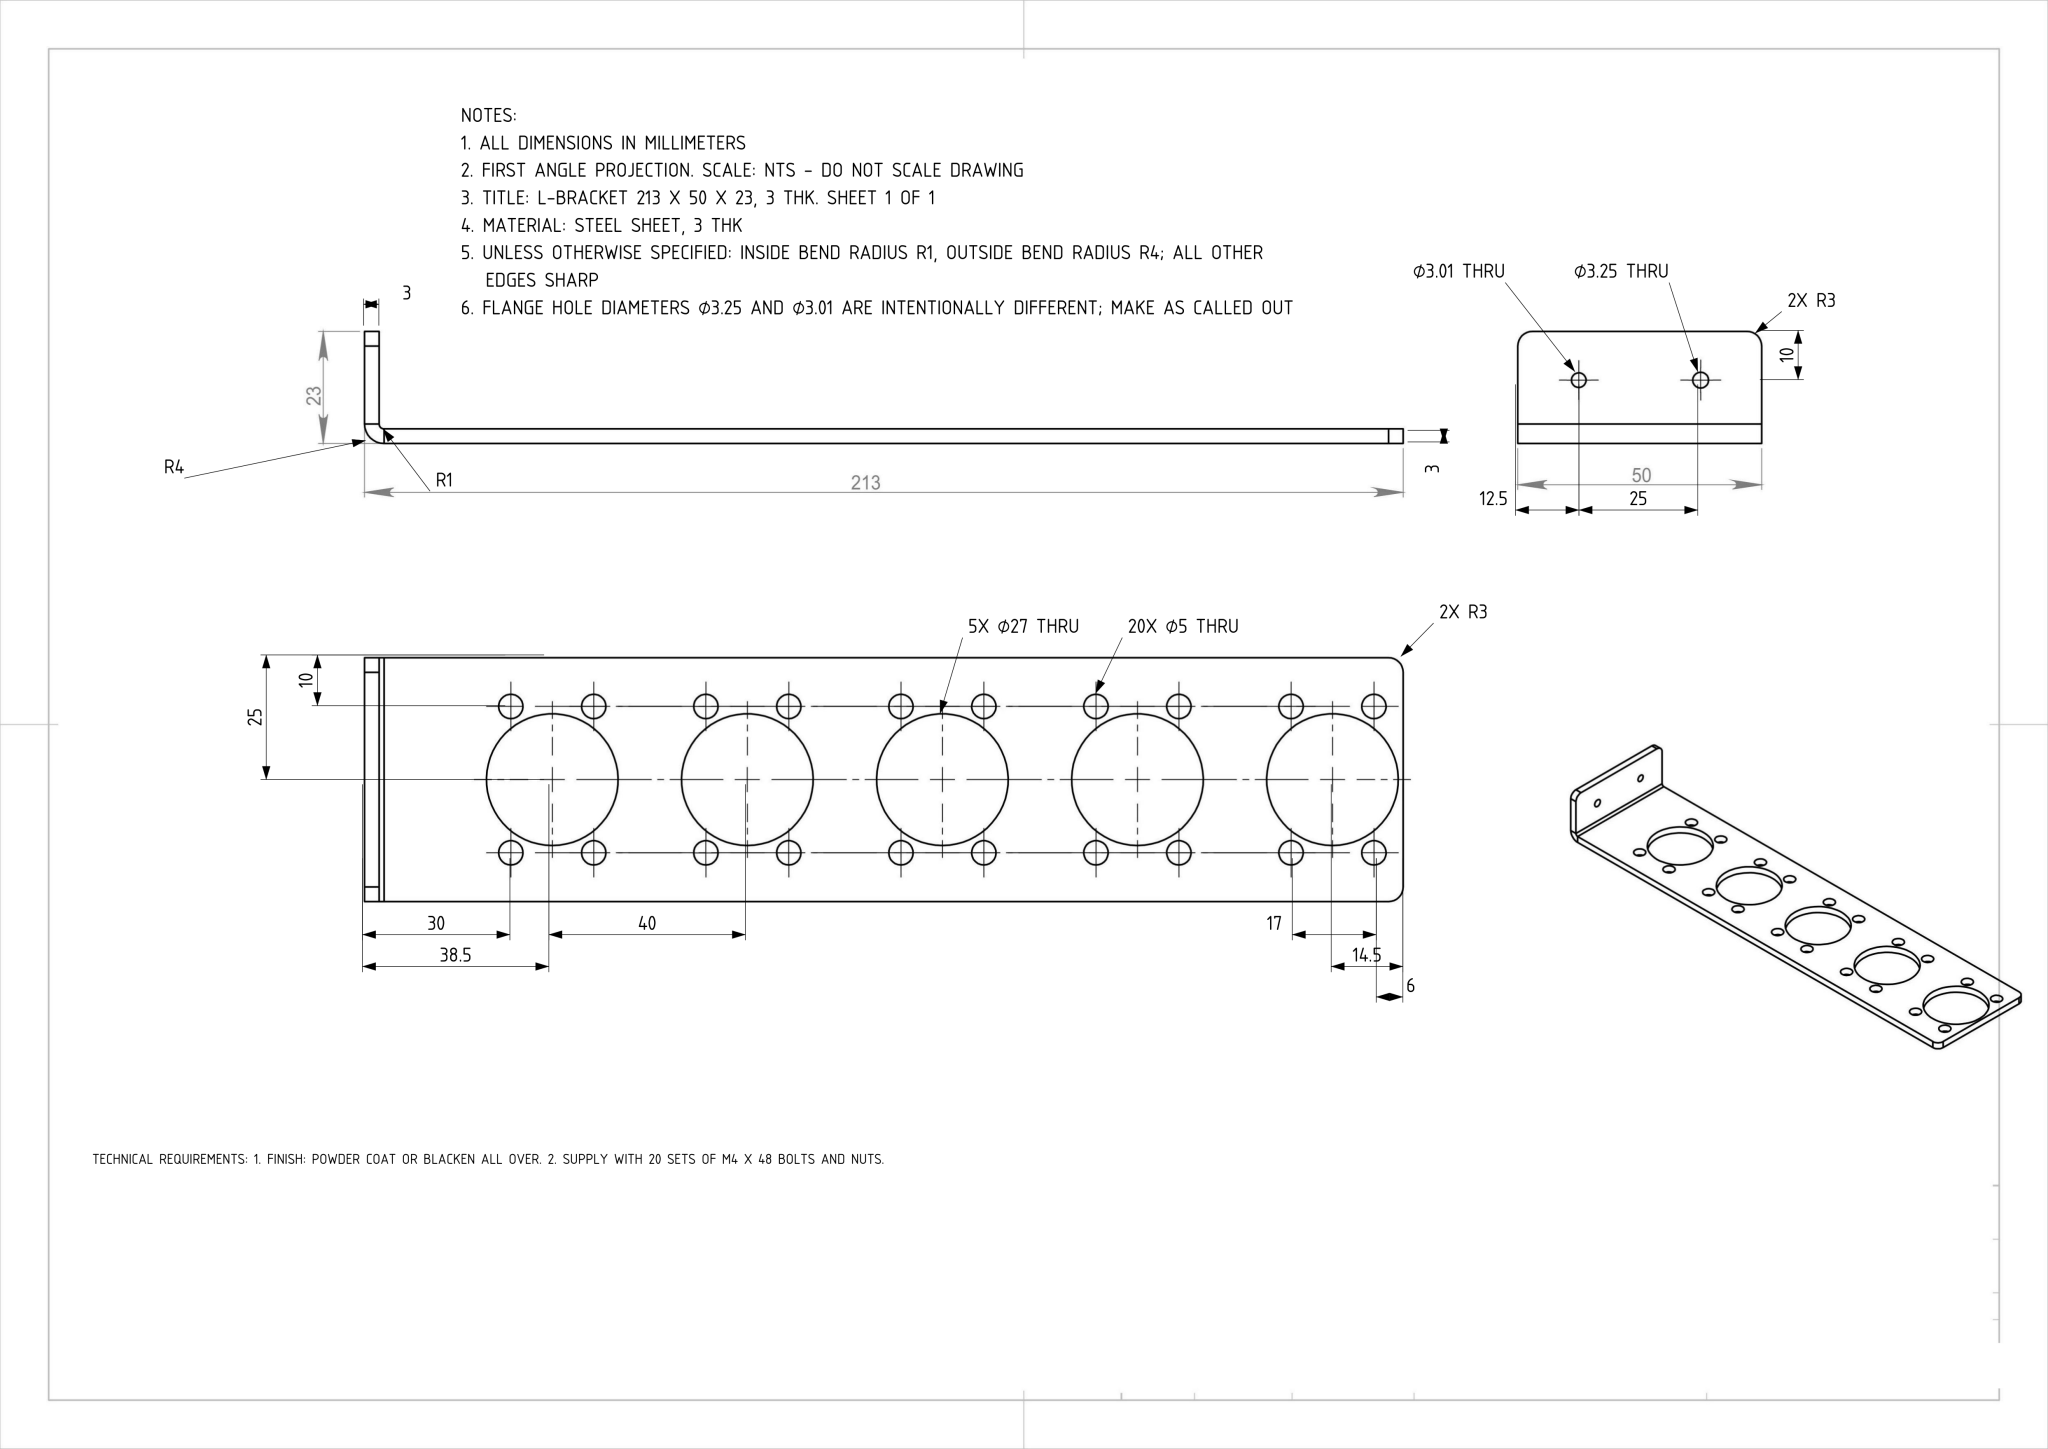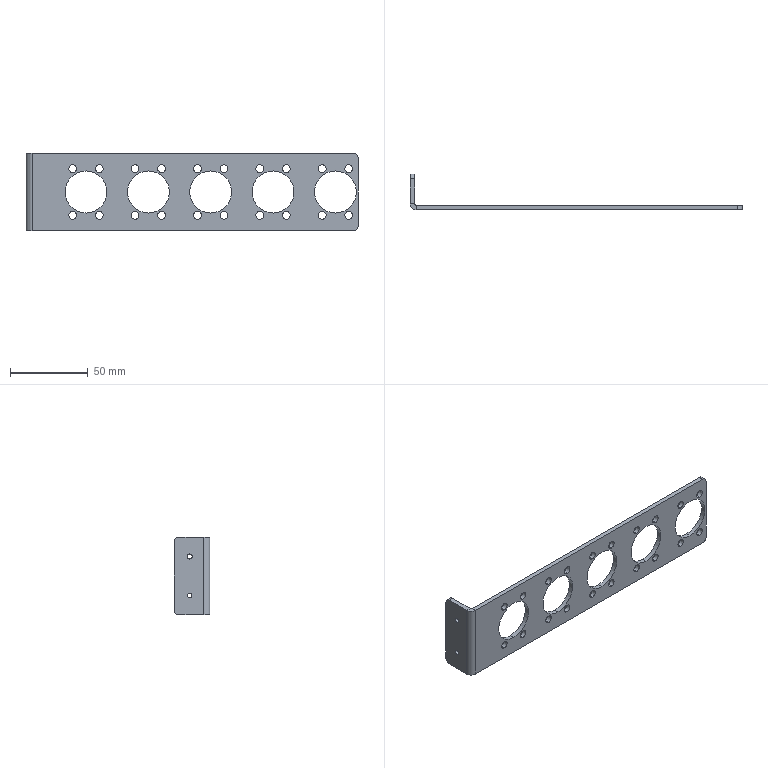Part | NX | mm | 1 solid | 72 faces | box 213 x 23 x 50 mm | volume 24953 mm3 | cylinder 60 | plane 12 | commonest cylinder face diameters 5 x40 27 x10 6 x4 3.251 x2 3.015 x2 2 x1 8 x1